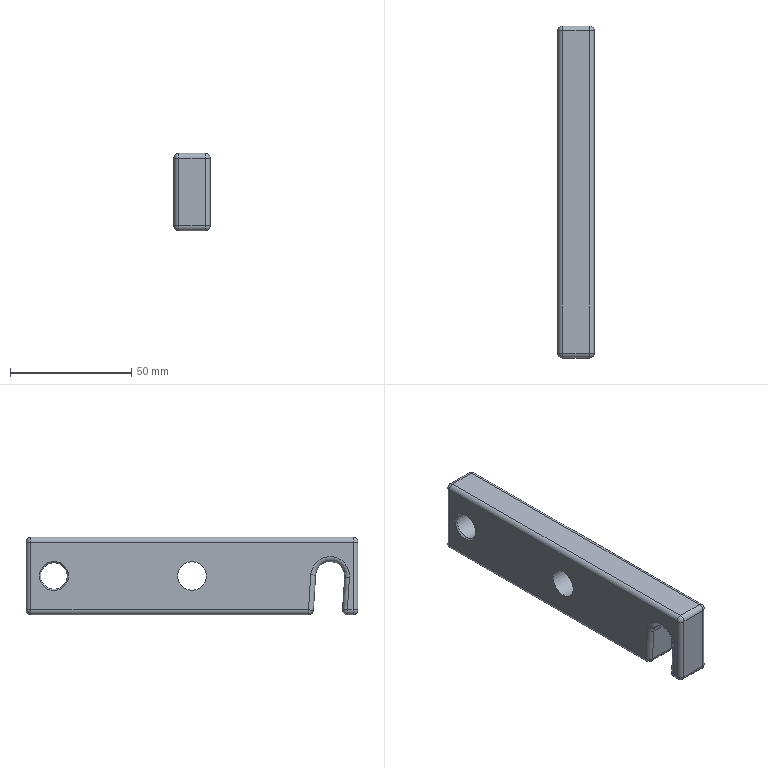Component | NX | CLAMP_PLATE | 1 solid | 47 faces | volume 58245 mm3 | cylinder 23 | sphere 12 | plane 9 | torus 2 | cone 1 | commonest cylinder face diameters 4 x20 12 x1 11 x1 11.8 x1